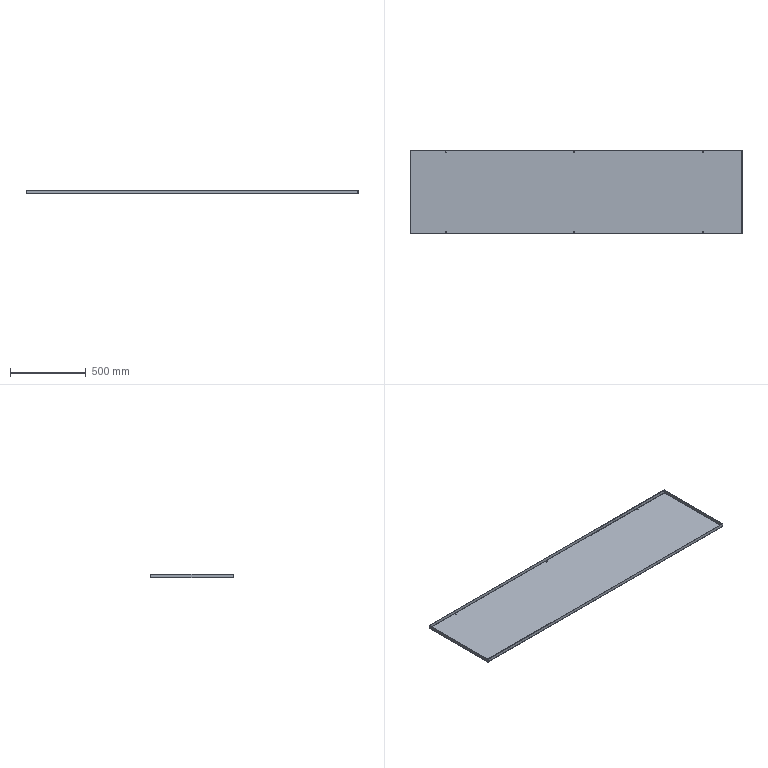Component | SolidWorks | SideDoorAssembly-1_SideDoorPG50-101-1 | 1 solid | 54 faces | volume 1970771 mm3 | plane 34 | cylinder 20 | commonest cylinder face diameters 6 x12 3.3 x4 0.3 x4 | material AISI 1045 Steel, cold drawn